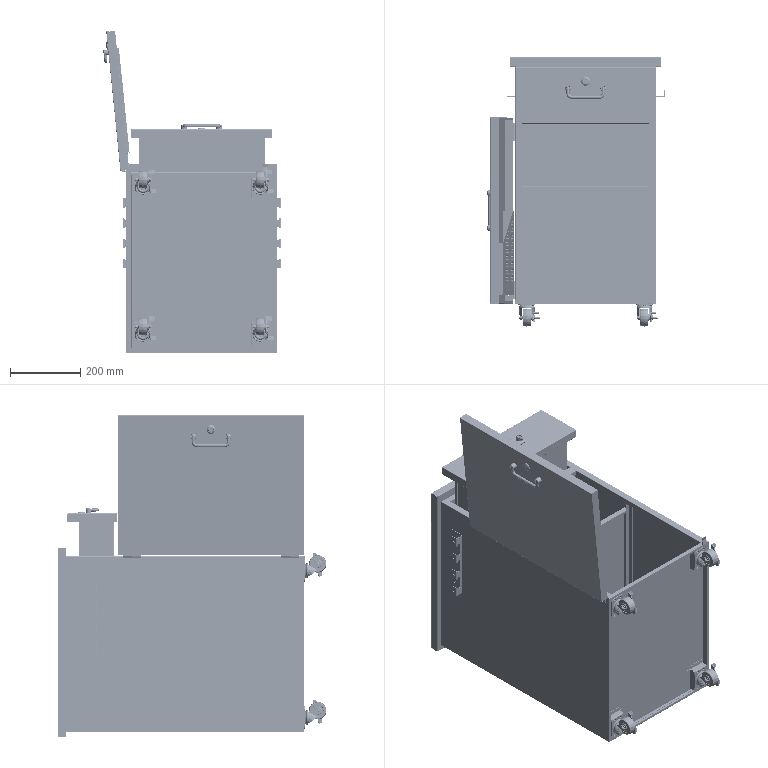Assembly | SolidWorks | mm | 42 component files | 54 solids | 4930 faces | box 504.7 x 764.51 x 918.14 mm | volume 3030700 mm3 | plane 1928 | cylinder 1918 | torus 468 | spline 370 | cone 126 | sphere 120 | commonest cylinder face diameters 5 x822 0.2 x120 18 x102 6 x98 2.2 x91 9.5 x44 3.2 x39 4 x36
Bill of materials:
2InchCaster | 4 |  | Swivel caster-like assembly: rectangular top plate with four corner holes, a ball-race style swivel ring, a U-shaped fork, a wide cylindrical wheel on a hex-nut axle, and a bent lever/tab mechanism on one side.
C1 | 4 |  | Cylindrical roller/wheel body with a concentric through-bore, a smaller raised hub boss on one face, and a recessed annular step around the boss.
C2 | 2 |  | U-shaped bent round rod with two parallel legs joined by a straight span, radiused bends, rounded leg ends and a small cross-hole near each leg tip.
DoorPanel | 1 | SPCC | Large shallow rectangular tray/panel with folded perimeter flanges forming a thin box lid. The face has one central larger hole with flats and two smaller round holes beside it.
Folder | 1 | SPCC | Sheet-metal side panel with a trapezoidal profile (one sloped edge), a dense grid of round perforations, and folded flanges/offset return along the straight vertical edge and top.
DrawerBackPanel | 1 | SPCC | Long flat rectangular sheet with a short downturned J-shaped hook/return along one long edge and small offset tabs at the ends.
DrawerBody | 1 | SPCC | U-channel sheet-metal panel: wide flat web with two perpendicular side walls, each ending in a small outward-turned lip.
DrawerFrontPanel | 1 | SPCC | Rectangular plate/thin box cover with one larger hole with flats and two smaller round holes on its top face, and short side walls around the perimeter.
HangingPlate | 2 | SUS201-Brushed | Bent sheet-metal bracket with an asymmetric U/J profile: one wide flange with two slotted/oval holes, and a narrower opposite flange cut into a series of notched tabs/hook teeth.
Imported1 | 2 |  | Hinge-leaf-like flat plate with a rolled cylindrical knuckle along part of one edge. The leaf has a stepped L-shaped outline, two through-holes, and three small dimples/holes near the knuckle.
Imported2 | 2 |  | Plain solid cylindrical pin/rod with small chamfers at the ends.
Imported3 | 2 |  | Hinge-leaf-like flat plate with a rolled open-curl knuckle along part of one edge. The leaf has an L-shaped/stepped outline and two round through-holes.
Lock1 | 2 | Ductile Iron | Hollow flanged cylindrical bushing with external helical-style ridges (thread-like) along the shank and a longitudinal flat cut along one side of the threaded section.
Lock3 | 2 |  | Thin obround (stadium-shaped) flat plate with a short solid cylindrical boss projecting from one face, placed off-center toward one end.
BottomPlate | 1 | SPCC | Thin flat rectangular sheet panel with a small bent hook or offset return formed along one long edge.
DoorSupport | 1 | SPCC | Narrow flat strip tab with one rounded end and a single round through-hole near that end, with two bends forming a joggled/angled profile.
FootPlate | 1 | SPCC | Bent sheet bracket: rectangular main plate with one large central round hole and four smaller holes in a rectangular pattern, with a flange bent off one edge that ends in an upturned lip giving a Z/step profile, plus a narrow side flange.
FootPlate2 | 1 | SPCC | Bent sheet bracket similar to the preceding one: rectangular plate with a large central hole and four smaller corner holes, with a top flange ending in an upturned lip and a perpendicular flange along one side, arranged mirror-wise.
FootPlate3 | 1 | SPCC | Bent sheet bracket with a rectangular hole-pattern plate (one large central hole, four smaller holes) and formed flanges along the side and bottom edges giving a Z/step profile.
FootPlate4 | 1 | SPCC | Bent sheet bracket with a rectangular plate carrying one large central hole and four smaller holes, with a bottom flange and an offset side flange, mirrored relative to unnamed part.
MainBody | 1 | SPCC | Open U-shaped sheet channel/tray: flat base with two tall parallel side walls, each ending in a small inward hook/return lip at the top, with a few small holes near one end of each wall.
MiddleBeam | 1 | SPCC | Long straight sheet channel with a C-type section: web and two legs with rounded bends, one leg carrying a short inward return lip so the open side is partially closed.
ShelfBeam | 2 | SPCC | Long straight angle (L-section) profile with a rounded inside/outside bend; one leg appears longer than the other.
SlideRailMountingPlate | 2 | SPCC | Long straight hat-section (omega) sheet profile: raised center web with two side walls and outward flanges at the base, with a few small holes along the web.
TopPlate | 1 | SPCC | Thin rectangular plate, slightly taller than wide, with a raised inner rectangular field on one face. The field has sloped or chamfered edges and sits inside a flat border around the outside.
UpperBeam | 1 | SPCC | Long straight profile with a constant, thin-walled bent cross-section. Starting at one end, the section has a short upstanding flange, a long flat web, a downturned leg, and a short return flange pointing back under the web. All bends are rounded.
Shelf | 1 | SPCC | Thin, plain, flat rectangular plate, nearly square, with no visible holes or surface features.
Mates:
1. coincident | MainBodyWeldment-1/FootPlate3-1 face at (-195.783, -328.128, 176.001) dir (0, -1, 0) | 2InchCaster-1 face at (-185.033, -328.128, 231.626) dir (0, 1, 0)
2. concentric | MainBodyWeldment-1/FootPlate3-1 face at (-182.703, -326.628, 182.066) dir (0, -1, 0) r 3 | 2InchCaster-1 face at (-182.703, -330.208, 182.066) dir (0, 1, 0) r 3.2
3. concentric | MainBodyWeldment-1/FootPlate3-1 face at (-182.703, -326.628, 235.936) dir (0, -1, 0) r 3 | 2InchCaster-1 face at (-182.703, -330.208, 235.936) dir (0, 1, 0) r 3.2
4. coincident | MainBodyWeldment-1/MainBody-1 face at (196.217, 371.872, -249.999) dir (1, 0, 0) | DrawerWelding-1/DrawerFrontPanel-1 face at (196.217, 2344.872, 348.252) dir (1, 0, 0)
5. distance | DrawerWelding-1/DrawerFrontPanel-1 face at (-2203.783, 344.872, 348.252) dir (0, 1, 0) | MainBodyWeldment-1/TopPlate-1 face at (-2533.783, 347.872, 275.001) dir (0, -1, 0)
6. coincident | MainBodyWeldment-1/MainBody-1 face at (-203.783, 371.872, 250.001) dir (-1, 0, 0) | HangingPlate-1 face at (-203.783, 261.872, 176.501) dir (1, 0, 0)
7. concentric | MainBodyWeldment-1/MainBody-1 face at (196.217, 291.872, 150.001) dir (-1, 0, 0) r 2.5 | HangingPlate-1 face at (-203.783, 291.872, 150.001) dir (-1, 0, 0) r 3.5
8. concentric | MainBodyWeldment-1/MainBody-1 face at (196.217, 291.872, 0.001262) dir (-1, 0, 0) r 2.5 | HangingPlate-1 face at (-203.783, 291.872, 0.001262) dir (-1, 0, 0) r 3.5
9. coincident | MainBodyWeldment-1/MainBody-1 face at (196.217, 371.872, -249.999) dir (1, 0, 0) | HangingPlate-2 face at (196.217, 261.872, -23.499) dir (-1, 0, 0)
10. concentric | MainBodyWeldment-1/MainBody-1 face at (196.217, 291.872, 150.001) dir (-1, 0, 0) r 2.5 | HangingPlate-2 face at (196.217, 291.872, 150.001) dir (1, 0, 0) r 3.5
11. concentric | MainBodyWeldment-1/MainBody-1 face at (196.217, 291.872, 0.001262) dir (-1, 0, 0) r 2.5 | HangingPlate-2 face at (196.217, 291.872, 0.001262) dir (1, 0, 0) r 3.5
12. concentric | Imported2-1 face at (-208.19, 187.272, 251.017) dir (0, -1, 0) r 2.375 | Imported3-1 face at (-208.19, 136.472, 251.017) dir (0, -1, 0) r 4.407
13. concentric | Imported1-1 face at (-208.19, 187.272, 251.017) dir (0, 1, 0) r 4.407 | Imported2-1 face at (-208.19, 187.272, 251.017) dir (0, -1, 0) r 2.375
14. coincident | Imported2-1 face at (-208.19, 187.272, 251.017) dir (0, 1, 0) | Imported3-1 face at (-208.19, 187.272, 251.017) dir (0, 1, 0)
15. coincident | Imported1-1 face at (-205.815, 187.272, 229.681) dir (0, 1, 0) | Imported3-1 face at (-208.19, 187.272, 251.017) dir (0, 1, 0)
16. coincident | MainBodyWeldment-1/MainBody-1 face at (-203.783, 371.872, 250.001) dir (-1, 0, 0) | Imported1-1 face at (-203.783, 136.472, 229.681) dir (1, 0, 0)
17. coincident | DoorPanelWelding-1/DoorPanel-1 face at (-210.741, 2851.872, 255.187) dir (0.1012, 0, -0.9949) | Imported3-1 face at (-229.862, 187.272, 253.242) dir (-0.1012, 0, 0.9949)
18. concentric | MainBodyWeldment-1/MainBody-1 face at (-202.783, 177.747, 237.301) dir (-1, 0, 0) r 2.422 | Imported1-1 face at (-203.783, 177.747, 237.301) dir (-1, 0, 0) r 2.642
19. concentric | MainBodyWeldment-1/MainBody-1 face at (-202.783, 145.997, 237.301) dir (-1, 0, 0) r 2.422 | Imported1-1 face at (-203.783, 145.997, 237.301) dir (-1, 0, 0) r 2.642
20. concentric | DoorPanelWelding-1/DoorPanel-1 face at (-222.382, 177.747, 255.008) dir (0.1012, 0, -0.9949) r 1.1 | Imported3-1 face at (-222.281, 177.747, 254.013) dir (0.1012, 0, -0.9949) r 2.642
21. concentric | DoorPanelWelding-1/DoorPanel-1 face at (-222.382, 145.997, 255.008) dir (0.1012, 0, -0.9949) r 1.1 | Imported3-1 face at (-222.281, 145.997, 254.013) dir (0.1012, 0, -0.9949) r 2.642
22. concentric | Imported3-2 face at (-208.19, -313.528, 251.017) dir (0, -1, 0) r 4.407 | Imported2-2 face at (-208.19, -262.728, 251.017) dir (0, -1, 0) r 2.375
23. coincident | Imported3-2 face at (-208.19, -262.728, 251.017) dir (0, 1, 0) | Imported2-2 face at (-208.19, -262.728, 251.017) dir (0, 1, 0)
24. concentric | Imported1-2 face at (-208.19, -262.728, 251.017) dir (0, 1, 0) r 4.407 | Imported2-2 face at (-208.19, -262.728, 251.017) dir (0, -1, 0) r 2.375
25. coincident | Imported3-2 edge at (-229.862, -262.728, 253.242) dir (0.9949, 0, 0.1012) | Imported1-2 face at (-205.815, -262.728, 229.681) dir (0, 1, 0)
26. coincident | MainBodyWeldment-1/MainBody-1 face at (-203.783, 371.872, 250.001) dir (-1, 0, 0) | Imported1-2 face at (-203.783, -313.528, 229.681) dir (1, 0, 0)
27. concentric | MainBodyWeldment-1/MainBody-1 face at (-202.783, -304.003, 237.301) dir (-1, 0, 0) r 2.422 | Imported1-2 face at (-203.783, -304.003, 237.301) dir (-1, 0, 0) r 2.642
28. concentric | MainBodyWeldment-1/MainBody-1 face at (-202.783, -272.253, 237.301) dir (-1, 0, 0) r 2.422 | Imported1-2 face at (-203.783, -272.253, 237.301) dir (-1, 0, 0) r 2.642
29. coincident | DoorPanelWelding-1/DoorPanel-1 face at (-210.741, 2851.872, 255.187) dir (0.1012, 0, -0.9949) | Imported3-2 face at (-229.862, -262.728, 253.242) dir (-0.1012, 0, 0.9949)
30. coincident | Lock1-1 face at (-251.059, -63.128, 612.944) dir (0.9949, 0, 0.1012) | Lock3-1 face at (-254.184, -60.296, 643.656) dir (-0.9949, 0, -0.1012)
31. concentric | Lock1-1 face at (-274.936, -63.128, 610.515) dir (0.9949, 0, 0.1012) r 7.5 | Lock3-1 face at (-259.018, -63.128, 612.134) dir (0.9949, 0, 0.1012) r 5
32. concentric | DoorPanelWelding-1/DoorPanel-1 face at (-269.962, -63.128, 611.021) dir (-0.9949, 0, -0.1012) r 9.9 | Lock3-1 face at (-251.059, -63.128, 612.944) dir (0.9949, 0, 0.1012) r 8
33. coincident | DoorPanelWelding-1/DoorPanel-1 face at (-234.518, -328.128, 252.768) dir (-0.9949, 0, -0.1012) | Lock1-1 face at (-270.956, -63.128, 610.919) dir (0.9949, 0, 0.1012)
34. coincident | DoorPanelWelding-1/DoorPanel-1 edge at (-270.475, -54.628, 616.07) dir (0.1012, 0, -0.9949) | Lock1-1 face at (-271.716, -54.628, 618.381) dir (0, 1, 0)
35. concentric | Lock1-2 face at (-3.783, 304.872, 376.152) dir (0, 0, -1) r 7.5 | Lock3-2 face at (-3.783, 304.872, 360.152) dir (0, 0, -1) r 5
36. coincident | Lock1-2 face at (-3.783, 304.872, 352.152) dir (0, 0, -1) | Lock3-2 face at (10.41, 332.432, 352.152) dir (0, 0, 1)
37. concentric | DrawerWelding-1/DrawerFrontPanel-1 face at (-3.783, 304.872, 371.152) dir (0, 0, 1) r 9.9 | Lock1-2 face at (-3.783, 304.872, 352.152) dir (0, 0, 1) r 9
38. coincident | DrawerWelding-1/DrawerFrontPanel-1 face at (-203.783, 204.872, 372.152) dir (0, 0, 1) | Lock1-2 face at (-3.783, 304.872, 372.152) dir (0, 0, -1)
39. coincident | DrawerWelding-1/DrawerFrontPanel-1 edge at (1.293, 313.372, 371.152) dir (-1, 0, 0) | Lock1-2 face at (3.717, 313.372, 372.152) dir (0, 1, 0)
40. concentric | DoorPanelWelding-1/DoorPanel-1 face at (-267.937, -13.128, 591.123) dir (-0.9949, 0, -0.1012) r 4.1 | C1-1/C1-2 face at (-266.942, -13.128, 591.225) dir (-0.9949, 0, -0.1012) r 4
41. concentric | DoorPanelWelding-1/DoorPanel-1 face at (-267.937, -113.128, 591.123) dir (-0.9949, 0, -0.1012) r 4.1 | C1-1/C1-1 face at (-266.942, -113.128, 591.225) dir (-0.9949, 0, -0.1012) r 4
42. coincident | DoorPanelWelding-1/DoorPanel-1 face at (-234.518, -328.128, 252.768) dir (-0.9949, 0, -0.1012) | C1-1/C1-1 face at (-268.932, -113.128, 591.022) dir (0.9949, 0, 0.1012)
43. concentric | DrawerWelding-1/DrawerFrontPanel-1 face at (-53.783, 284.872, 371.152) dir (0, 0, 1) r 4.1 | C1-2/C1-2 face at (-53.783, 284.872, 370.152) dir (0, 0, 1) r 4
44. coincident | DrawerWelding-1/DrawerFrontPanel-1 face at (-203.783, 204.872, 372.152) dir (0, 0, 1) | C1-2/C1-2 face at (-53.783, 284.872, 372.152) dir (0, 0, -1)
45. concentric | DrawerWelding-1/DrawerFrontPanel-1 face at (46.217, 284.872, 371.152) dir (0, 0, 1) r 4.1 | C1-2/C1-1 face at (46.217, 284.872, 370.152) dir (0, 0, 1) r 4
46. coincident | MainBodyWeldment-1/ShelfBeam-2 face at (195.217, -8.128, -248.999) dir (0, 1, 0) | Shelf-1 face at (192.217, -8.128, -2147.942) dir (0, -1, 0)
47. distance | Shelf-1 face at (192.217, -7.028, -2147.942) dir (1, 0, 0) | MainBodyWeldment-1/MainBody-1 face at (196.217, 371.872, -249.999) dir (1, 0, 0)
48. concentric | C2-1 face at (-76.18, 13.703, -12.25) dir (1, 0, 0) r 2 | C1-1 face at (-79.68, 13.703, -12.25) dir (1, 0, 0) r 2.5
49. concentric | C2-1 face at (-76.18, 13.703, -12.25) dir (1, 0, 0) r 2 | C1-2 face at (20.32, 13.703, -12.25) dir (1, 0, 0) r 2.5
50. distance | C1-2 plane at (28.32, 8.708, -12.047) dir (1, 0, 0) | C1-1 plane at (-71.68, 8.708, -12.047) dir (1, 0, 0)
51. coincident | C2-1 plane at (-71.68, 13.703, -17.25) dir (1, 0, 0) | C1-1 plane at (-71.68, 8.708, -12.047) dir (1, 0, 0)
52. coincident | C1-1 face at (-71.68, 22.696, -12.616) dir (0, 0.9992, -0.04066) | C1-2 face at (28.32, 22.696, -12.616) dir (0, 0.9992, -0.04066)
53. coincident | DoorPanel-1 face at (-307.537, -260.805, 6.499) dir (0, 0, -1) | Folder-1 face at (-266.537, -235.805, 6.499) dir (0, 0, 1)
54. distance | Folder-1 face at (42.463, 14.195, -23.501) dir (1, 0, 0) | DoorPanel-1 face at (92.463, -2910.805, -16.401) dir (1, 0, 0)
55. distance | Folder-1 face at (-266.537, -235.805, 5.499) dir (0, -1, 0) | DoorPanel-1 face at (-2957.537, -260.805, -16.401) dir (0, -1, 0)
56. coincident | DrawerBody-1 face at (122.913, -54.468, -393.5) dir (0, 0, -1) | DrawerBackPanel-1 face at (131.913, -55.568, -393.5) dir (0, 0, 1)
57. coincident | DrawerBody-1 face at (121.913, 44.432, 6.5) dir (0, 1, 0) | DrawerBackPanel-1 face at (131.913, 44.432, -393.5) dir (0, 1, 0)
58. coincident | DrawerBody-1 face at (131.913, 44.432, 6.5) dir (1, 0, 0) | DrawerBackPanel-1 face at (131.913, 43.332, -394.5) dir (1, 0, 0)
59. coincident | DrawerFrontPanel-1 face at (-247.087, -63.568, 6.5) dir (0, 0, -1) | DrawerBody-1 face at (-217.087, -54.468, 6.5) dir (0, 0, 1)
60. coincident | DrawerFrontPanel-1 face at (2152.913, -55.568, -17.5) dir (0, 1, 0) | DrawerBody-1 face at (-216.087, -55.568, 6.5) dir (0, -1, 0)
61. distance | DrawerBody-1 face at (122.913, -54.568, 6.5) dir (1, 0, 0) | DrawerFrontPanel-1 face at (152.913, 2076.432, -16.4) dir (1, 0, 0)
62. distance | BottomPlate-1 face at (64.146, -333.5, 200) dir (1, 0, 0) | MainBody-1 face at (64.396, 366.5, -300) dir (-1, 0, 0)
63. coincident | MainBody-1 face at (-334.604, -333.5, 200) dir (0, 0, 1) | BottomPlate-1 face at (64.146, -333.5, 200) dir (0, 0, 1)
64. coincident | MainBody-1 face at (-334.604, -333.5, 200) dir (0, -1, 0) | BottomPlate-1 face at (64.146, -333.5, 192) dir (0, -1, 0)
65. coincident | MainBody-1 face at (-334.604, -333.5, 200) dir (0, 0, 1) | UpperBeam-1 face at (45.396, 326.5, 200) dir (0, 0, 1)
66. coincident | MainBody-1 face at (-334.604, -333.5, 200) dir (0, 0, 1) | MiddleBeam-1 face at (45.396, 179.5, 200) dir (0, 0, 1)
67. distance | MiddleBeam-1 face at (45.396, 204.5, 200) dir (0, 1, 0) | UpperBeam-1 face at (45.396, 326.5, 200) dir (0, -1, 0)
68. coincident | MainBody-1 face at (-334.604, 366.5, 200) dir (-1, 0, 0) | TopPlate-1 face at (-334.604, 342.5, -2630) dir (1, 0, 0)
69. coincident | MainBody-1 face at (-334.604, 366.5, -300) dir (0, 0, -1) | TopPlate-1 face at (2395.396, 342.5, -300) dir (0, 0, 1)
70. coincident | MainBody-1 face at (-334.604, 366.5, 200) dir (0, 1, 0) | TopPlate-1 face at (52.324, 366.5, 2540) dir (0, -1, 0)
71. coincident | MainBody-1 face at (45.396, -333.5, 200) dir (-1, 0, 0) | MiddleBeam-1 face at (45.396, 203.4, 199) dir (1, 0, 0)
72. coincident | BottomPlate-1 face at (64.146, -314.5, 185) dir (0, -1, 0) | FootPlate-1 face at (7.396, -314.5, -226) dir (0, 1, 0)
73. coincident | MainBody-1 face at (64.296, -333.5, -292) dir (0, 0, 1) | FootPlate-1 face at (8.896, -331.9, -292) dir (0, 0, -1)
74. coincident | MainBody-1 face at (57.396, -333.5, 191.75) dir (-1, 0, 0) | FootPlate-1 face at (57.396, -332, -226) dir (1, 0, 0)
75. coincident | MainBody-1 face at (64.296, -333.5, -292) dir (0, 0, 1) | FootPlate2-1 face at (-276.504, -316.1, -292) dir (0, 0, -1)
76. coincident | MainBody-1 face at (-326.604, -333.5, 191.75) dir (1, 0, 0) | FootPlate2-1 face at (-326.604, -332, -292) dir (-1, 0, 0)
77. coincident | MainBody-1 face at (-334.604, -333.5, 200) dir (0, -1, 0) | FootPlate2-1 face at (-326.604, -333.5, -292) dir (0, -1, 0)
78. coincident | BottomPlate-1 face at (64.146, -314.5, 185) dir (0, -1, 0) | FootPlate3-1 face at (-326.604, -314.5, 192) dir (0, 1, 0)
79. coincident | MainBody-1 face at (-326.604, -333.5, 191.75) dir (1, 0, 0) | FootPlate3-1 face at (-326.604, -332, 126) dir (-1, 0, 0)
80. coincident | BottomPlate-1 face at (64.146, -332.5, 192) dir (0, 0, -1) | FootPlate3-1 face at (-278.104, -331.9, 192) dir (0, 0, 1)
81. coincident | MainBody-1 face at (57.396, -333.5, 191.75) dir (-1, 0, 0) | FootPlate4-1 face at (57.396, -332, 192) dir (1, 0, 0)
82. coincident | BottomPlate-1 face at (64.146, -332.5, 192) dir (0, 0, -1) | FootPlate4-1 face at (7.296, -316.1, 192) dir (0, 0, 1)
83. coincident | BottomPlate-1 face at (64.146, -333.5, 192) dir (0, -1, 0) | FootPlate4-1 face at (57.396, -333.5, 192) dir (0, -1, 0)
84. coincident | MainBody-1 face at (-333.604, 366.5, 200) dir (1, 0, 0) | SlideRailMountingPlate-1 face at (-333.604, 268.645, -278) dir (-1, 0, 0)
85. coincident | MainBody-1 edge at (-314.604, 354.5, 185) dir (0, -1, 0) | SlideRailMountingPlate-1 face at (-332.004, 270.145, 185) dir (0, 0, 1)
86. coincident | MainBody-1 face at (64.396, 366.5, -300) dir (-1, 0, 0) | SlideRailMountingPlate-2 face at (64.396, 259.645, -278) dir (1, 0, 0)
87. coincident | MainBody-1 edge at (45.396, -321.25, 185) dir (0, 1, 0) | SlideRailMountingPlate-2 face at (46.996, 270.145, 185) dir (0, 0, 1)
88. coincident | SlideRailMountingPlate-1 face at (-332.104, 298.645, -278) dir (0, 1, 0) | SlideRailMountingPlate-2 face at (45.396, 298.645, -278) dir (0, 1, 0)
89. coincident | BottomPlate-1 face at (64.146, -333.5, 192) dir (0, -1, 0) | DoorSupport-1 face at (55.396, -333.5, 199.993) dir (0, 1, 0)
90. distance | DoorSupport-1 face at (55.396, -334.986, 200.198) dir (1, 0, 0) | MainBody-1 face at (65.396, 366.5, -300) dir (1, 0, 0)
91. coincident | BottomPlate-1 face at (64.146, -333.5, 200) dir (0, 0, 1) | DoorSupport-1 edge at (55.396, -333.499, 200) dir (-1, 0, 0)
92. coincident | MainBody-1 face at (-333.604, 366.5, 200) dir (1, 0, 0) | ShelfBeam-1 face at (-333.604, -28.5, 186) dir (-1, 0, 0)
93. coincident | MainBody-1 face at (-334.604, 366.5, -299) dir (0, 0, 1) | ShelfBeam-1 face at (-332.004, -15, -299) dir (0, 0, -1)
94. coincident | MainBody-1 face at (64.396, 366.5, -300) dir (-1, 0, 0) | ShelfBeam-2 face at (64.396, -28.5, -299) dir (1, 0, 0)
95. coincident | MainBody-1 face at (-334.604, 366.5, -299) dir (0, 0, 1) | ShelfBeam-2 edge at (62.896, -28.5, -299) dir (0, 1, 0)
96. coincident | ShelfBeam-1 face at (-333.604, -13.5, 186) dir (0, 1, 0) | ShelfBeam-2 face at (64.396, -13.5, -299) dir (0, 1, 0)
97. distance | ShelfBeam-1 face at (-333.604, -13.5, 186) dir (0, 1, 0) | BottomPlate-1 face at (64.146, -313.5, 185) dir (0, 1, 0)
98. coincident | UpperBeam-1 face at (45.396, 366.5, 200) dir (0, 1, 0) | TopPlate-1 face at (-2664.604, 366.5, 196.928) dir (0, -1, 0)
99. coincident | MainBody-1 face at (45.396, -333.5, 200) dir (-1, 0, 0) | UpperBeam-1 face at (45.396, 327.6, 198.9) dir (1, 0, 0)